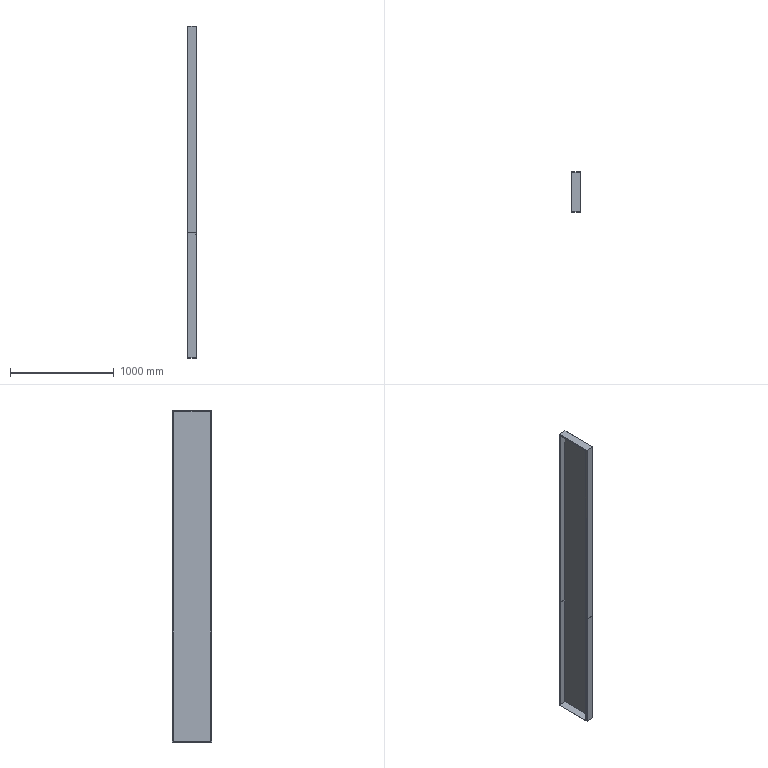Component | NX | CB3 | 1 solid | 30 faces | volume 2798222 mm3 | plane 30